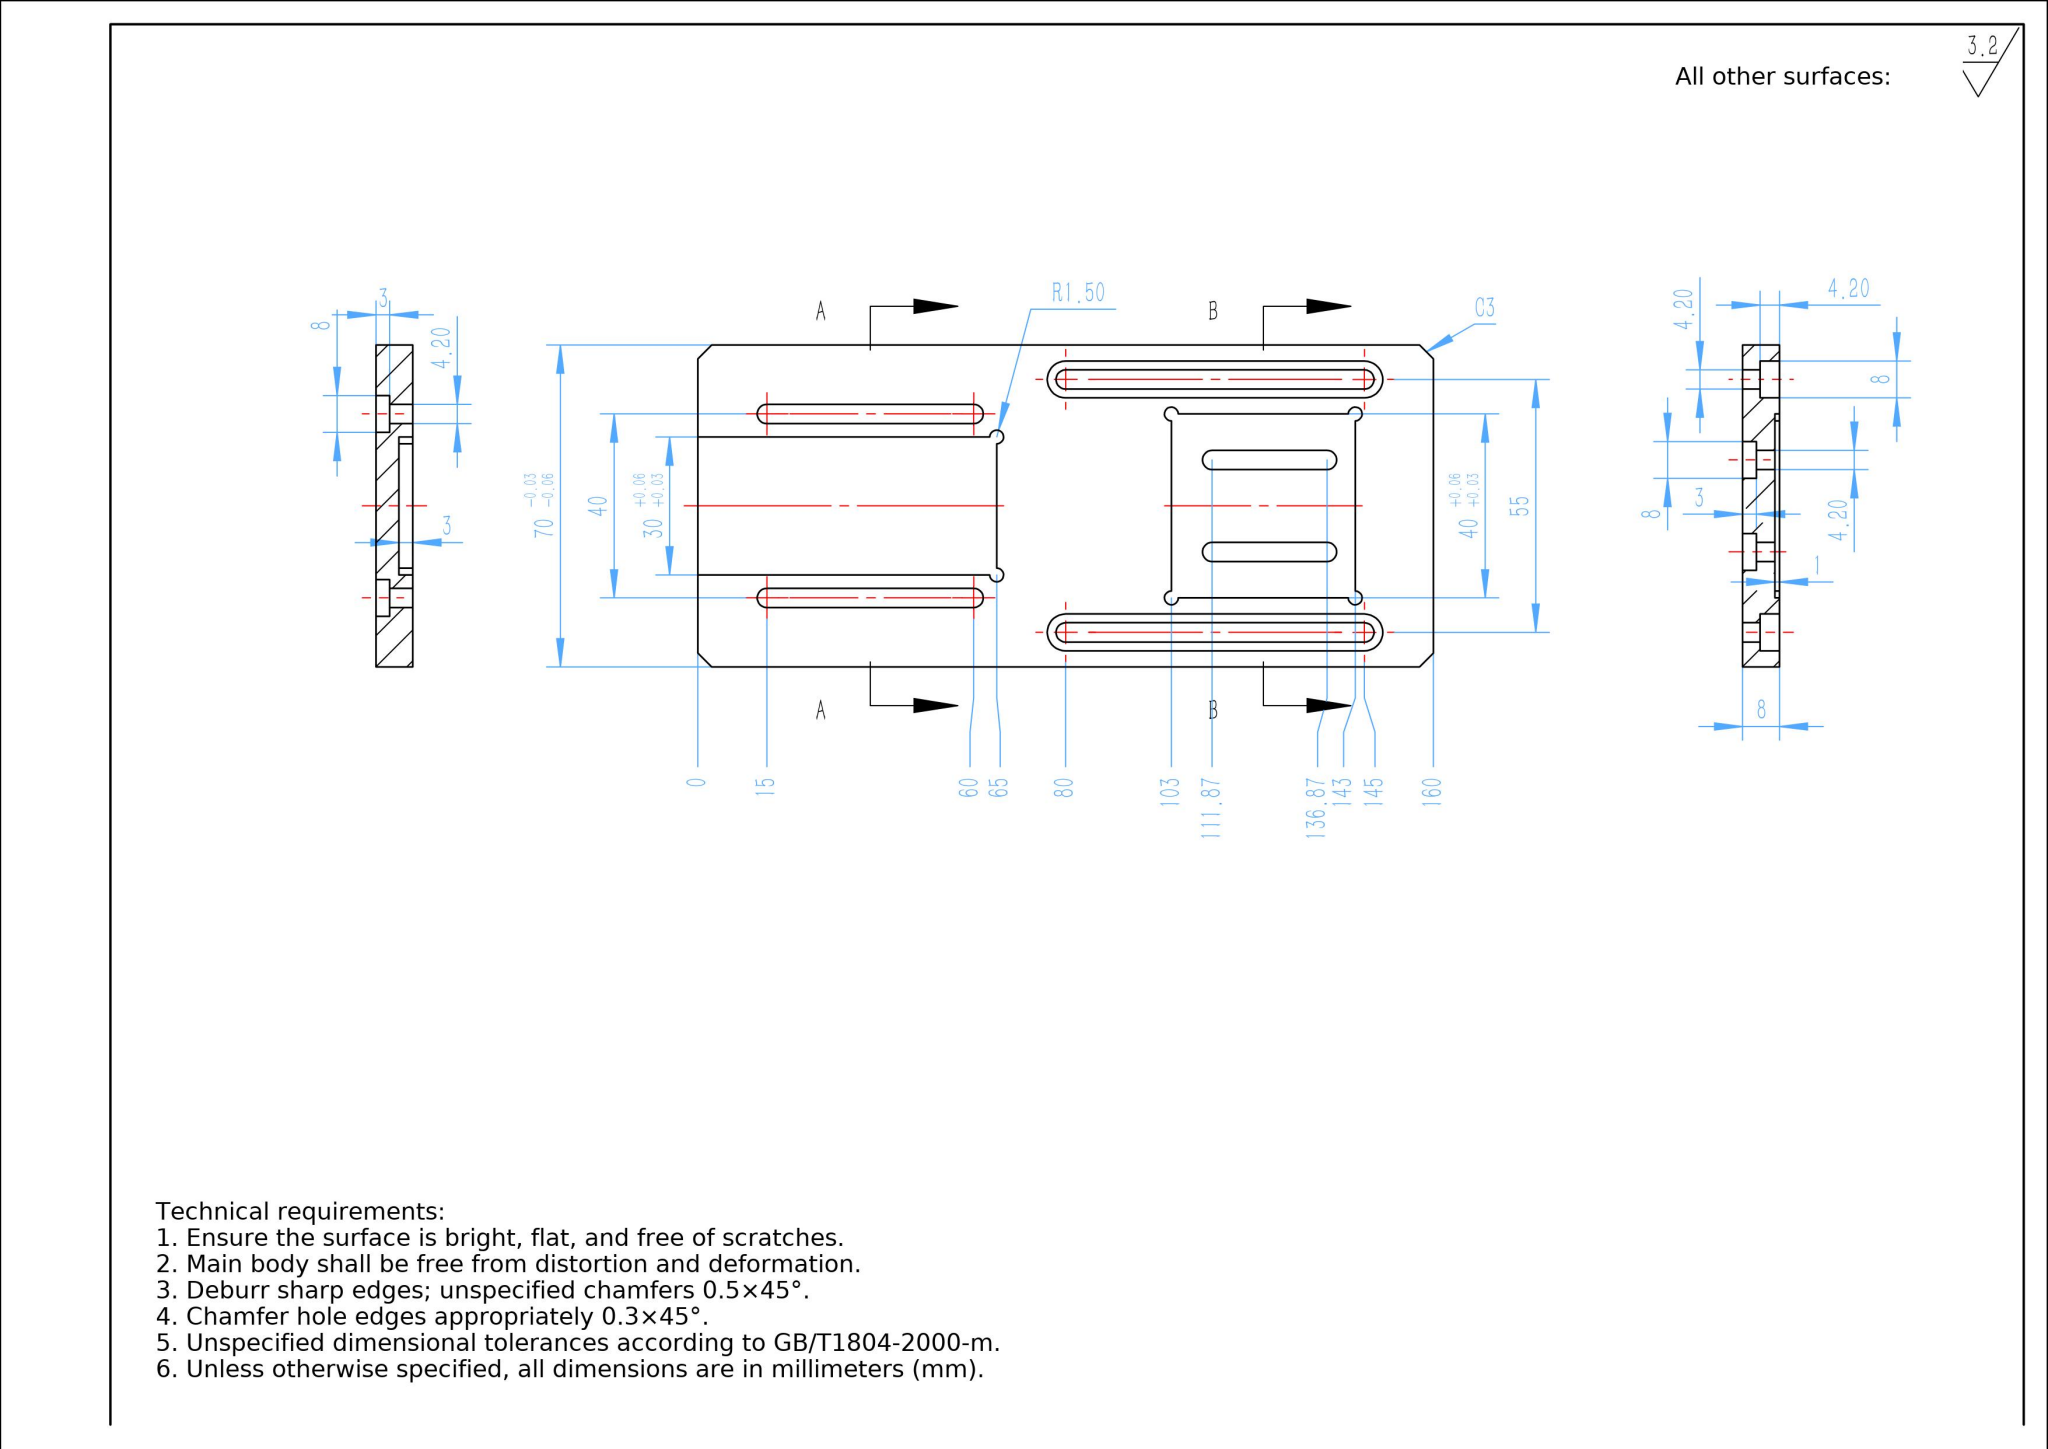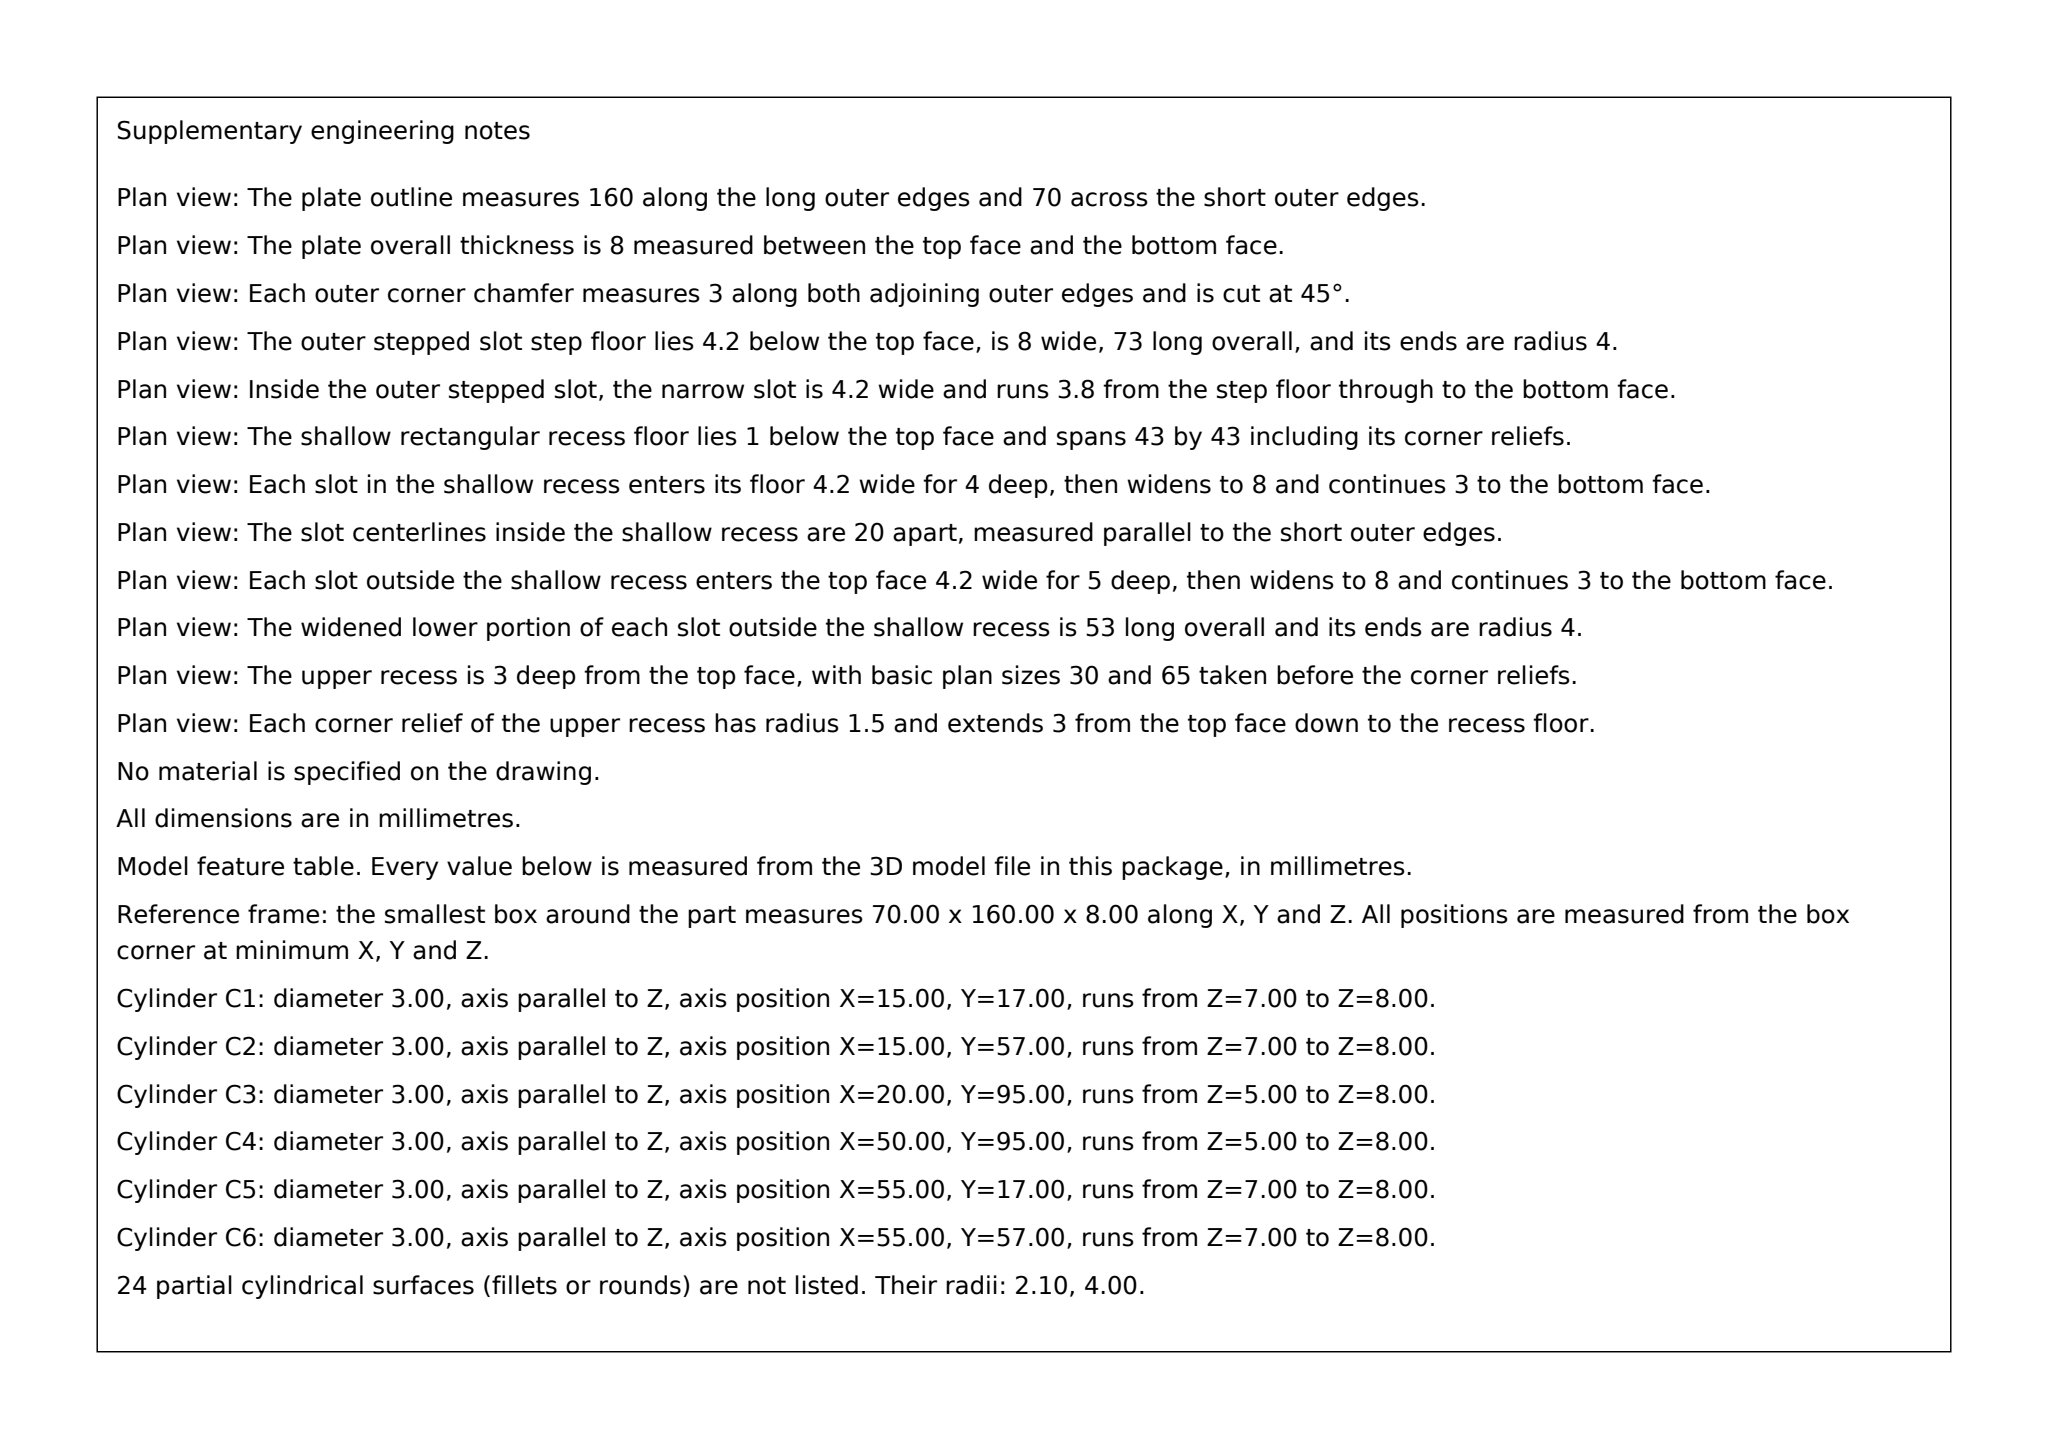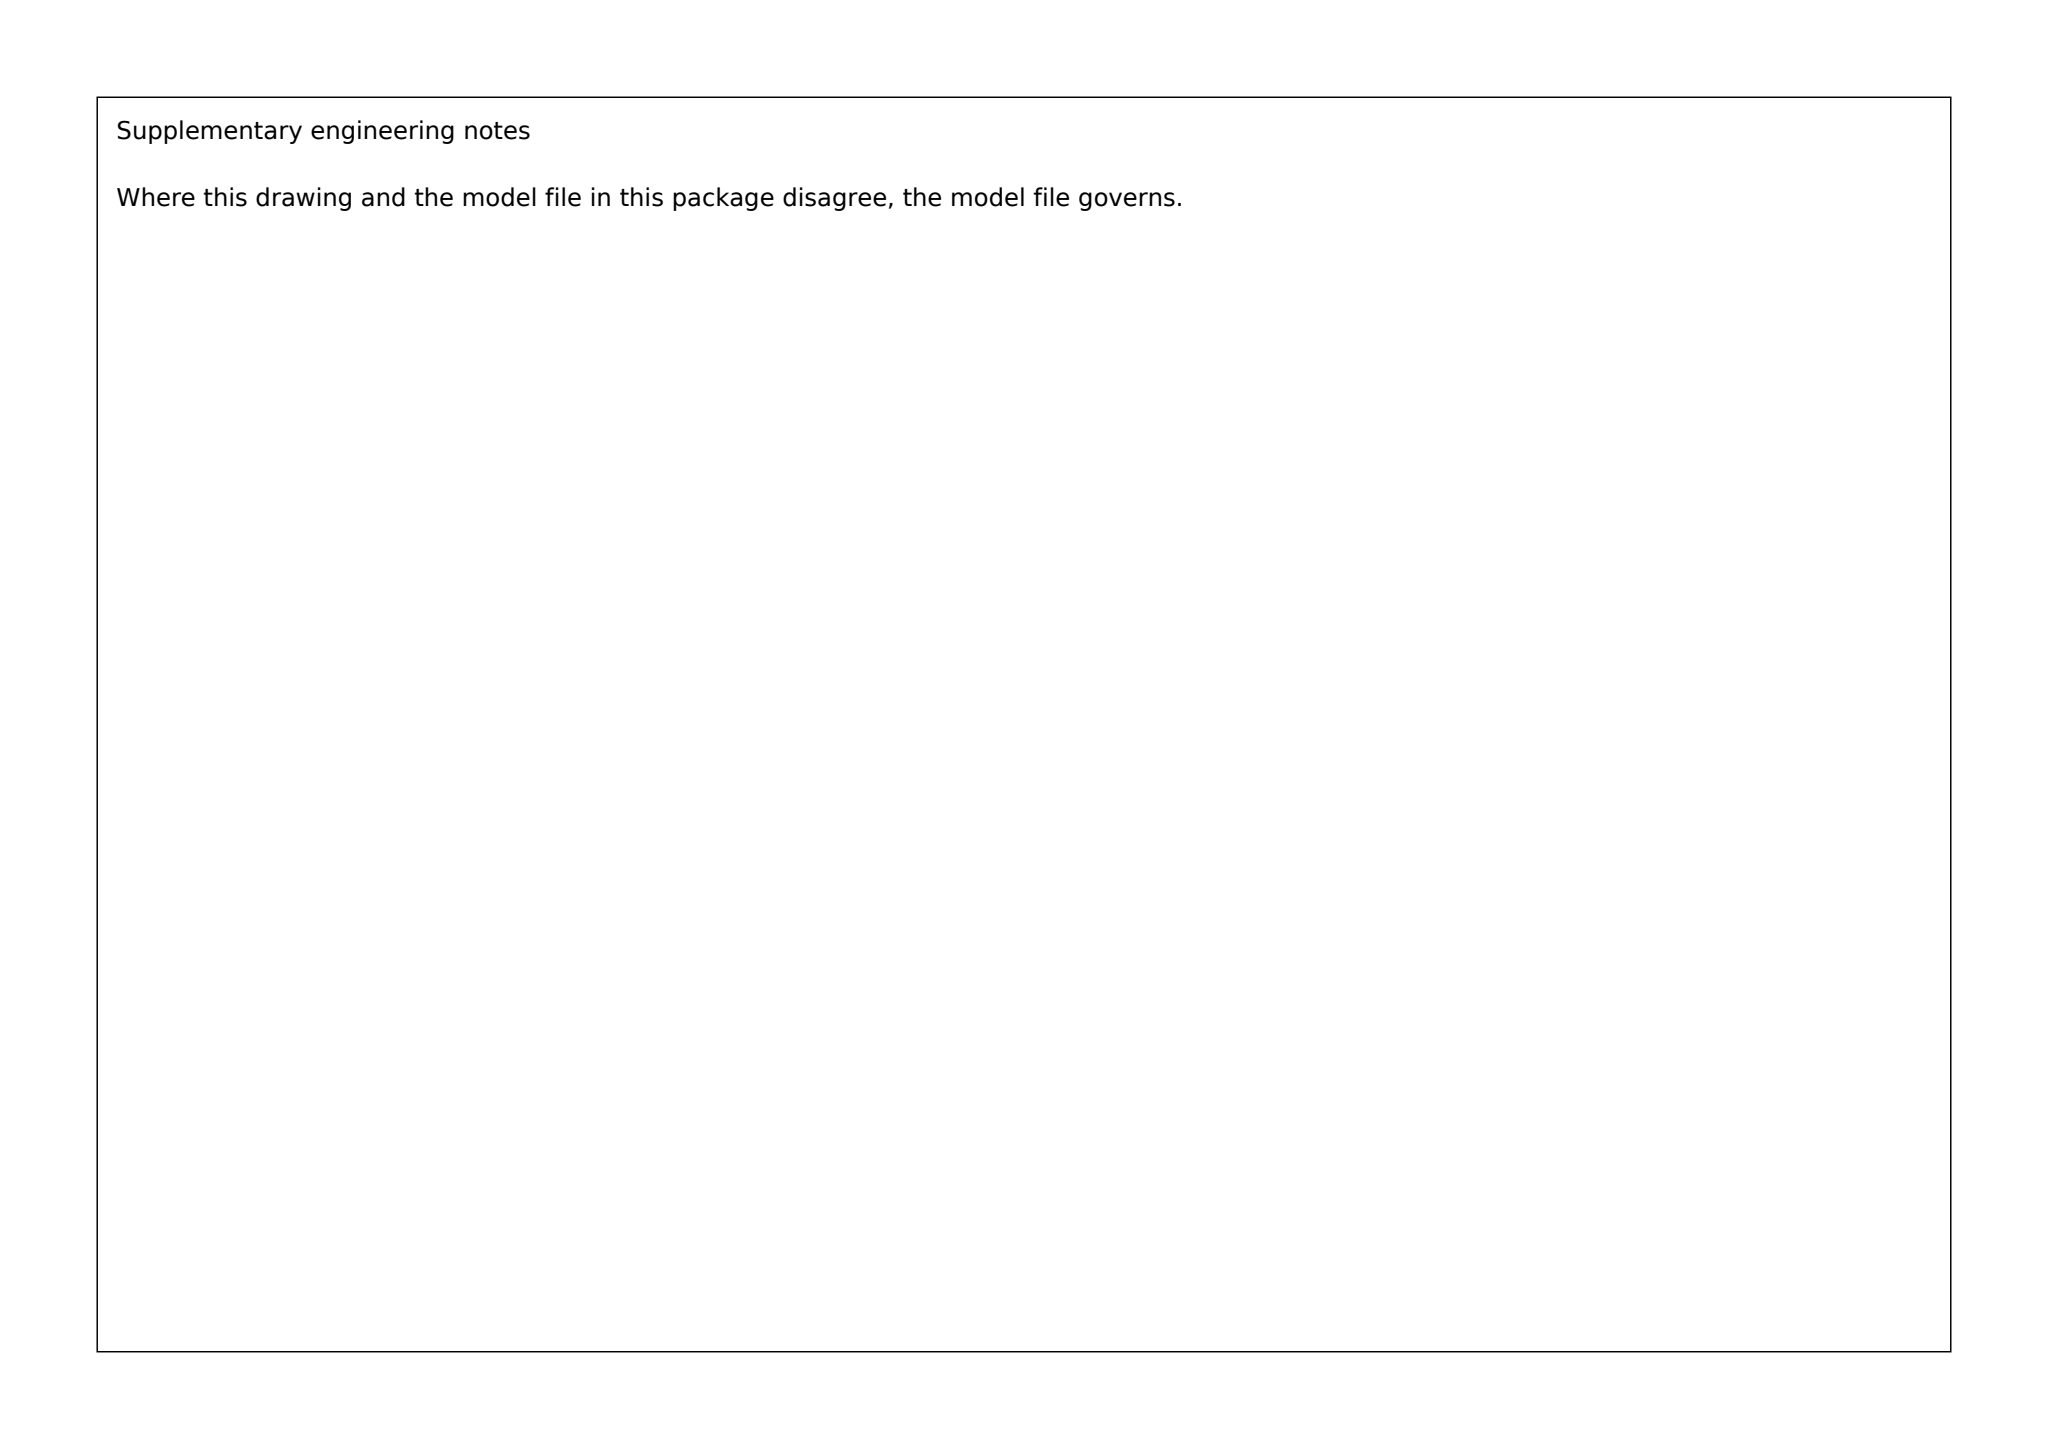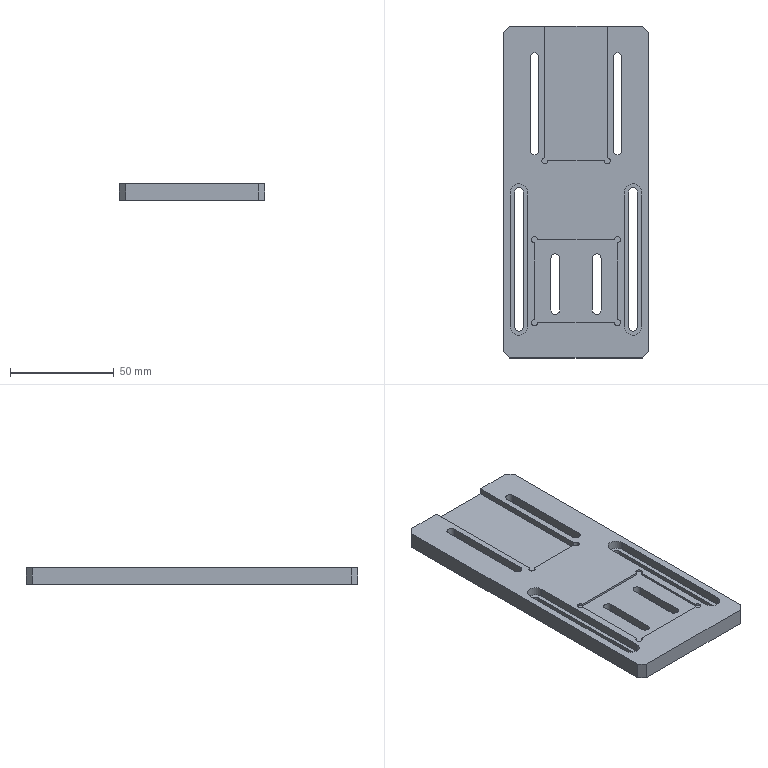Part | SolidWorks | mm | 1 solid | 82 faces | box 70 x 160 x 8 mm | volume 68040 mm3 | plane 49 | cylinder 33 | commonest cylinder face diameters 4.2 x12 8 x12 3 x9
build123d program:
from build123d import *

# Parameters (mm, degrees)
SKETCH1_W           = 70
SKETCH1_H           = 160
BOSS_EXTRUDE1_DEPTH = 8
SKETCH2_W           = 30
SKETCH2_H           = 65
CUT_EXTRUDE1_DEPTH  = 3
SKETCH3_W           = 40
SKETCH3_H           = 40
CUT_EXTRUDE2_DEPTH  = 1
CUT_EXTRUDE3_DEPTH  = 4.2
CUT_EXTRUDE4_DEPTH  = 88.422
CUT_EXTRUDE5_DEPTH  = 88.687
CUT_EXTRUDE6_DEPTH  = 3
CUT_EXTRUDE7_DEPTH  = 3
CUT_EXTRUDE8_DEPTH  = 88.464
CHAMFER1_SIZE       = 3
SKETCH10_R          = 1.5
CUT_EXTRUDE9_DEPTH  = 88.601
SKETCH11_R          = 1.5
CUT_EXTRUDE10_DEPTH = 88.464


with BuildPart() as part:
    # Sketch1 → Boss-Extrude1 (new body)
    with BuildSketch(Plane.XY):
        Rectangle(SKETCH1_W, SKETCH1_H)
    extrude(amount=-BOSS_EXTRUDE1_DEPTH)

    # Sketch2 → Cut-Extrude1 (cut)
    with BuildSketch(Plane.XY):
        with Locations((0, 47.5)):
            Rectangle(SKETCH2_W, SKETCH2_H)
    extrude(amount=-CUT_EXTRUDE1_DEPTH, mode=Mode.SUBTRACT)

    # Sketch3 → Cut-Extrude2 (cut)
    with BuildSketch(Plane.XY):
        with Locations((0, -43)):
            Rectangle(SKETCH3_W, SKETCH3_H)
    extrude(amount=-CUT_EXTRUDE2_DEPTH, mode=Mode.SUBTRACT)

    # Sketch4 → Cut-Extrude3 (cut)
    with BuildSketch(Plane.XY):
        with BuildLine():
            Line((-23.5, 0), (-23.5, -65))
            ThreePointArc((-23.5, -65), (-27.5, -69), (-31.5, -65))
            Line((-31.5, -65), (-31.5, 0))
            ThreePointArc((-31.5, 0), (-27.5, 4), (-23.5, 0))
        make_face()
    cut_extrude3 = extrude(amount=-CUT_EXTRUDE3_DEPTH, mode=Mode.SUBTRACT)

    # Sketch5 → Cut-Extrude4 (cut, through all)
    with BuildSketch(Plane.XY.offset(-4.2)):
        with BuildLine():
            Line((-25.4, 0), (-25.4, -65))
            ThreePointArc((-25.4, -65), (-27.5, -67.1), (-29.6, -65))
            Line((-29.6, -65), (-29.6, 0))
            ThreePointArc((-29.6, 0), (-27.5, 2.1), (-25.4, 0))
        make_face()
    cut_extrude4 = extrude(amount=-CUT_EXTRUDE4_DEPTH, mode=Mode.SUBTRACT)

    # Sketch6 → Cut-Extrude5 (cut, through all)
    with BuildSketch(Plane.XY):
        with BuildLine():
            Line((-17.9, 65), (-17.9, 20))
            ThreePointArc((-17.9, 20), (-20, 17.9), (-22.1, 20))
            Line((-22.1, 20), (-22.1, 65))
            ThreePointArc((-22.1, 65), (-20, 67.1), (-17.9, 65))
        make_face()
    cut_extrude5 = extrude(amount=-CUT_EXTRUDE5_DEPTH, mode=Mode.SUBTRACT)

    # Sketch7 → Cut-Extrude6 (cut)
    with BuildSketch(Plane(origin=(0, 0, -8), x_dir=(-1, 0, 0), z_dir=(0, 0, -1))):
        with BuildLine():
            Line((24, 65), (24, 20))
            ThreePointArc((24, 20), (20, 16), (16, 20))
            Line((16, 20), (16, 65))
            ThreePointArc((16, 65), (20, 69), (24, 65))
        make_face()
    cut_extrude6 = extrude(amount=-CUT_EXTRUDE6_DEPTH, mode=Mode.SUBTRACT)

    # Mirror1: Cut-Extrude3, Cut-Extrude4, Cut-Extrude5, Cut-Extrude6 across plane
    add(cut_extrude3.mirror(Plane(origin=(0, 0, 0), x_dir=(0, 0, 1), z_dir=(1, 0, 0))), mode=Mode.SUBTRACT)
    add(cut_extrude4.mirror(Plane(origin=(0, 0, 0), x_dir=(0, 0, 1), z_dir=(1, 0, 0))), mode=Mode.SUBTRACT)
    add(cut_extrude5.mirror(Plane(origin=(0, 0, 0), x_dir=(0, 0, 1), z_dir=(1, 0, 0))), mode=Mode.SUBTRACT)
    add(cut_extrude6.mirror(Plane(origin=(0, 0, 0), x_dir=(0, 0, 1), z_dir=(1, 0, 0))), mode=Mode.SUBTRACT)

    # Sketch8 → Cut-Extrude7 (cut)
    with BuildSketch(Plane(origin=(0, 0, -8), x_dir=(-1, 0, 0), z_dir=(0, 0, -1))):
        with BuildLine():
            Line((-14, -56.87), (-14, -31.87))
            ThreePointArc((-14, -31.87), (-10, -27.87), (-6, -31.87))
            Line((-6, -31.87), (-6, -56.87))
            ThreePointArc((-6, -56.87), (-10, -60.87), (-14, -56.87))
        make_face()
    cut_extrude7 = extrude(amount=-CUT_EXTRUDE7_DEPTH, mode=Mode.SUBTRACT)

    # Sketch9 → Cut-Extrude8 (cut, through all)
    with BuildSketch(Plane(origin=(0, 0, -5), x_dir=(-1, 0, 0), z_dir=(0, 0, -1))):
        with BuildLine():
            Line((-7.9, -31.87), (-7.9, -56.87))
            ThreePointArc((-7.9, -56.87), (-10, -58.97), (-12.1, -56.87))
            Line((-12.1, -56.87), (-12.1, -31.87))
            ThreePointArc((-12.1, -31.87), (-10, -29.77), (-7.9, -31.87))
        make_face()
    cut_extrude8 = extrude(amount=-CUT_EXTRUDE8_DEPTH, mode=Mode.SUBTRACT)

    # Chamfer1
    chamfer1_edges = [part.edges().sort_by_distance(p)[0] for p in [
        (35, -80, -4),
        (-35, -80, -4),
        (-35, 80, -4),
        (35, 80, -4),
    ]]
    chamfer(chamfer1_edges, length=CHAMFER1_SIZE)

    # Sketch10 → Cut-Extrude9 (cut, through all)
    with BuildSketch(Plane.XY.offset(-1)):
        with Locations((-20, -23)):
            Circle(SKETCH10_R)
        with Locations((20, -23)):
            Circle(SKETCH10_R)
        with Locations((-20, -63)):
            Circle(SKETCH10_R)
        with Locations((20, -63)):
            Circle(SKETCH10_R)
    extrude(amount=CUT_EXTRUDE9_DEPTH, mode=Mode.SUBTRACT)

    # Sketch11 → Cut-Extrude10 (cut, through all)
    with BuildSketch(Plane.XY.offset(-3)):
        with Locations((-15, 15)):
            Circle(SKETCH11_R)
        with Locations((15, 15)):
            Circle(SKETCH11_R)
    extrude(amount=CUT_EXTRUDE10_DEPTH, mode=Mode.SUBTRACT)

    # Mirror2: Cut-Extrude7, Cut-Extrude8 across plane
    add(cut_extrude7.mirror(Plane(origin=(0, 0, 0), x_dir=(0, 0, 1), z_dir=(1, 0, 0))), mode=Mode.SUBTRACT)
    add(cut_extrude8.mirror(Plane(origin=(0, 0, 0), x_dir=(0, 0, 1), z_dir=(1, 0, 0))), mode=Mode.SUBTRACT)


solid = part.part